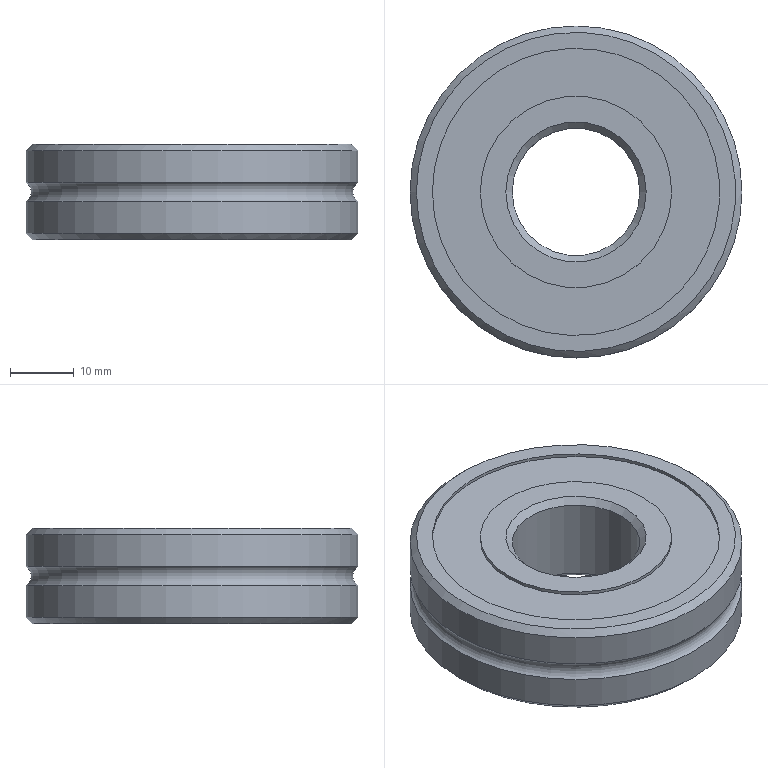Component | NX | BENT_SHAFT_2 | 1 solid | 18 faces | box 52 x 52 x 15 mm | volume 25760 mm3 | cylinder 7 | plane 6 | cone 4 | torus 1 | commonest cylinder face diameters 45 x2 30 x2 52 x2 20 x1
STEP:
#1=CARTESIAN_POINT('',(0.,0.,0.));
#2=DIRECTION('',(0.,0.,1.));
#3=DIRECTION('',(1.,0.,0.));
#4=AXIS2_PLACEMENT_3D('',#1,#2,#3);
#5=CARTESIAN_POINT('',(1437.632,1212.,804.574));
#6=VERTEX_POINT('',#5);
#7=CARTESIAN_POINT('',(1460.132,1212.,804.574));
#8=DIRECTION('',(0.,0.,-1.));
#9=DIRECTION('',(-1.,0.,0.));
#10=AXIS2_PLACEMENT_3D('',#7,#8,#9);
#11=CIRCLE('',#10,22.5);
#12=CARTESIAN_POINT('',(1435.132,1212.,804.574));
#13=DIRECTION('',(0.,0.,1.));
#14=DIRECTION('',(1.,0.,0.));
#15=AXIS2_PLACEMENT_3D('',#12,#13,#14);
#16=PLANE('',#15);
#17=CARTESIAN_POINT('',(2.5,0.));
#18=CARTESIAN_POINT('',(2.5,38.971));
#19=CARTESIAN_POINT('',(36.25,19.486));
#20=CARTESIAN_POINT('',(70.,0.));
#21=CARTESIAN_POINT('',(36.25,-19.486));
#22=CARTESIAN_POINT('',(2.5,-38.971));
#23=CARTESIAN_POINT('',(2.5,0.));
#24=(BOUNDED_CURVE()B_SPLINE_CURVE(2,(#17,#18,#19,#20,#21,#22,#23),.UNSPECIFIED.,.T.,.F.)B_SPLINE_CURVE_WITH_KNOTS((1,2,2,2,2,1),(-2.094,0.,2.094,4.189,6.283,8.378),.UNSPECIFIED.)CURVE()GEOMETRIC_REPRESENTATION_ITEM()RATIONAL_B_SPLINE_CURVE((1.,0.5,1.,0.5,1.,0.5,1.))REPRESENTATION_ITEM(''));
#25=(GEOMETRIC_REPRESENTATION_CONTEXT(2)PARAMETRIC_REPRESENTATION_CONTEXT()REPRESENTATION_CONTEXT('',''));
#26=DEFINITIONAL_REPRESENTATION('',(#24),#25);
#27=PCURVE('',#16,#26);
#28=CARTESIAN_POINT('',(1460.132,1212.,786.574));
#29=DIRECTION('',(0.,0.,-1.));
#30=DIRECTION('',(-1.,0.,0.));
#31=AXIS2_PLACEMENT_3D('',#28,#29,#30);
#32=CYLINDRICAL_SURFACE('',#31,22.5);
#33=CARTESIAN_POINT('',(0.,-18.));
#34=DIRECTION('',(1.,0.));
#35=VECTOR('',#34,1.);
#36=LINE('',#33,#35);
#37=(GEOMETRIC_REPRESENTATION_CONTEXT(2)PARAMETRIC_REPRESENTATION_CONTEXT()REPRESENTATION_CONTEXT('',''));
#38=DEFINITIONAL_REPRESENTATION('',(#36),#37);
#39=PCURVE('',#32,#38);
#40=SURFACE_CURVE('',#11,(#27,#39),.PCURVE_S1.);
#41=EDGE_CURVE('',#6,#6,#40,.T.);
#42=ORIENTED_EDGE('',*,*,#41,.F.);
#43=EDGE_LOOP('',(#42));
#44=FACE_BOUND('',#43,.T.);
#45=CARTESIAN_POINT('',(1435.132,1212.,804.574));
#46=VERTEX_POINT('',#45);
#47=CARTESIAN_POINT('',(1460.132,1212.,804.574));
#48=DIRECTION('',(0.,0.,-1.));
#49=DIRECTION('',(-1.,0.,0.));
#50=AXIS2_PLACEMENT_3D('',#47,#48,#49);
#51=CIRCLE('',#50,25.);
#52=CARTESIAN_POINT('',(0.,0.));
#53=CARTESIAN_POINT('',(0.,43.301));
#54=CARTESIAN_POINT('',(37.5,21.651));
#55=CARTESIAN_POINT('',(75.,0.));
#56=CARTESIAN_POINT('',(37.5,-21.651));
#57=CARTESIAN_POINT('',(0.,-43.301));
#58=CARTESIAN_POINT('',(0.,0.));
#59=(BOUNDED_CURVE()B_SPLINE_CURVE(2,(#52,#53,#54,#55,#56,#57,#58),.UNSPECIFIED.,.T.,.F.)B_SPLINE_CURVE_WITH_KNOTS((1,2,2,2,2,1),(-2.094,0.,2.094,4.189,6.283,8.378),.UNSPECIFIED.)CURVE()GEOMETRIC_REPRESENTATION_ITEM()RATIONAL_B_SPLINE_CURVE((1.,0.5,1.,0.5,1.,0.5,1.))REPRESENTATION_ITEM(''));
#60=(GEOMETRIC_REPRESENTATION_CONTEXT(2)PARAMETRIC_REPRESENTATION_CONTEXT()REPRESENTATION_CONTEXT('',''));
#61=DEFINITIONAL_REPRESENTATION('',(#59),#60);
#62=PCURVE('',#16,#61);
#63=CARTESIAN_POINT('',(1460.132,1212.,805.574));
#64=DIRECTION('',(0.,0.,1.));
#65=DIRECTION('',(1.,0.,0.));
#66=AXIS2_PLACEMENT_3D('',#63,#64,#65);
#67=CONICAL_SURFACE('',#66,26.,0.7854);
#68=CARTESIAN_POINT('',(9.425,-1.));
#69=DIRECTION('',(-1.,0.));
#70=VECTOR('',#69,1.);
#71=LINE('',#68,#70);
#72=(GEOMETRIC_REPRESENTATION_CONTEXT(2)PARAMETRIC_REPRESENTATION_CONTEXT()REPRESENTATION_CONTEXT('',''));
#73=DEFINITIONAL_REPRESENTATION('',(#71),#72);
#74=PCURVE('',#67,#73);
#75=SURFACE_CURVE('',#51,(#62,#74),.PCURVE_S1.);
#76=EDGE_CURVE('',#46,#46,#75,.T.);
#77=ORIENTED_EDGE('',*,*,#76,.T.);
#78=EDGE_LOOP('',(#77));
#79=FACE_BOUND('',#78,.T.);
#80=ADVANCED_FACE('',(#44,#79),#16,.F.);
#81=CARTESIAN_POINT('',(1437.632,1212.,805.074));
#82=VERTEX_POINT('',#81);
#83=CARTESIAN_POINT('',(1460.132,1212.,805.074));
#84=DIRECTION('',(0.,0.,-1.));
#85=DIRECTION('',(-1.,0.,0.));
#86=AXIS2_PLACEMENT_3D('',#83,#84,#85);
#87=CIRCLE('',#86,22.5);
#88=CARTESIAN_POINT('',(0.,-18.5));
#89=DIRECTION('',(1.,0.));
#90=VECTOR('',#89,1.);
#91=LINE('',#88,#90);
#92=(GEOMETRIC_REPRESENTATION_CONTEXT(2)PARAMETRIC_REPRESENTATION_CONTEXT()REPRESENTATION_CONTEXT('',''));
#93=DEFINITIONAL_REPRESENTATION('',(#91),#92);
#94=PCURVE('',#32,#93);
#95=CARTESIAN_POINT('',(1437.632,1212.,805.074));
#96=DIRECTION('',(0.,0.,1.));
#97=DIRECTION('',(1.,0.,0.));
#98=AXIS2_PLACEMENT_3D('',#95,#96,#97);
#99=PLANE('',#98);
#100=CARTESIAN_POINT('',(0.,0.));
#101=CARTESIAN_POINT('',(0.,38.971));
#102=CARTESIAN_POINT('',(33.75,19.486));
#103=CARTESIAN_POINT('',(67.5,0.));
#104=CARTESIAN_POINT('',(33.75,-19.486));
#105=CARTESIAN_POINT('',(0.,-38.971));
#106=CARTESIAN_POINT('',(0.,0.));
#107=(BOUNDED_CURVE()B_SPLINE_CURVE(2,(#100,#101,#102,#103,#104,#105,#106),.UNSPECIFIED.,.T.,.F.)B_SPLINE_CURVE_WITH_KNOTS((1,2,2,2,2,1),(-2.094,0.,2.094,4.189,6.283,8.378),.UNSPECIFIED.)CURVE()GEOMETRIC_REPRESENTATION_ITEM()RATIONAL_B_SPLINE_CURVE((1.,0.5,1.,0.5,1.,0.5,1.))REPRESENTATION_ITEM(''));
#108=(GEOMETRIC_REPRESENTATION_CONTEXT(2)PARAMETRIC_REPRESENTATION_CONTEXT()REPRESENTATION_CONTEXT('',''));
#109=DEFINITIONAL_REPRESENTATION('',(#107),#108);
#110=PCURVE('',#99,#109);
#111=SURFACE_CURVE('',#87,(#94,#110),.PCURVE_S1.);
#112=EDGE_CURVE('',#82,#82,#111,.T.);
#113=ORIENTED_EDGE('',*,*,#112,.T.);
#114=CARTESIAN_POINT('',(1437.632,1212.,805.074));
#115=CARTESIAN_POINT('',(1437.632,1212.,804.574));
#116=B_SPLINE_CURVE_WITH_KNOTS('',1,(#114,#115),.UNSPECIFIED.,.F.,.F.,(2,2),(-18.5,-18.),.PIECEWISE_BEZIER_KNOTS.);
#117=CARTESIAN_POINT('',(6.283,0.));
#118=DIRECTION('',(0.,1.));
#119=VECTOR('',#118,1.);
#120=LINE('',#117,#119);
#121=(GEOMETRIC_REPRESENTATION_CONTEXT(2)PARAMETRIC_REPRESENTATION_CONTEXT()REPRESENTATION_CONTEXT('',''));
#122=DEFINITIONAL_REPRESENTATION('',(#120),#121);
#123=PCURVE('',#32,#122);
#124=CARTESIAN_POINT('',(0.,0.));
#125=DIRECTION('',(0.,1.));
#126=VECTOR('',#125,1.);
#127=LINE('',#124,#126);
#128=(GEOMETRIC_REPRESENTATION_CONTEXT(2)PARAMETRIC_REPRESENTATION_CONTEXT()REPRESENTATION_CONTEXT('',''));
#129=DEFINITIONAL_REPRESENTATION('',(#127),#128);
#130=PCURVE('',#32,#129);
#131=SEAM_CURVE('',#116,(#123,#130),.PCURVE_S1.);
#132=EDGE_CURVE('',#82,#6,#131,.T.);
#133=ORIENTED_EDGE('',*,*,#132,.T.);
#134=ORIENTED_EDGE('',*,*,#41,.F.);
#135=ORIENTED_EDGE('',*,*,#132,.F.);
#136=EDGE_LOOP('',(#113,#133,#134,#135));
#137=FACE_BOUND('',#136,.F.);
#138=ADVANCED_FACE('',(#137),#32,.F.);
#139=CARTESIAN_POINT('',(1445.132,1212.,805.074));
#140=VERTEX_POINT('',#139);
#141=CARTESIAN_POINT('',(1460.132,1212.,805.074));
#142=DIRECTION('',(0.,0.,-1.));
#143=DIRECTION('',(-1.,0.,0.));
#144=AXIS2_PLACEMENT_3D('',#141,#142,#143);
#145=CIRCLE('',#144,15.);
#146=CARTESIAN_POINT('',(7.5,0.));
#147=CARTESIAN_POINT('',(7.5,25.981));
#148=CARTESIAN_POINT('',(30.,12.99));
#149=CARTESIAN_POINT('',(52.5,0.));
#150=CARTESIAN_POINT('',(30.,-12.99));
#151=CARTESIAN_POINT('',(7.5,-25.981));
#152=CARTESIAN_POINT('',(7.5,0.));
#153=(BOUNDED_CURVE()B_SPLINE_CURVE(2,(#146,#147,#148,#149,#150,#151,#152),.UNSPECIFIED.,.T.,.F.)B_SPLINE_CURVE_WITH_KNOTS((1,2,2,2,2,1),(-2.094,0.,2.094,4.189,6.283,8.378),.UNSPECIFIED.)CURVE()GEOMETRIC_REPRESENTATION_ITEM()RATIONAL_B_SPLINE_CURVE((1.,0.5,1.,0.5,1.,0.5,1.))REPRESENTATION_ITEM(''));
#154=(GEOMETRIC_REPRESENTATION_CONTEXT(2)PARAMETRIC_REPRESENTATION_CONTEXT()REPRESENTATION_CONTEXT('',''));
#155=DEFINITIONAL_REPRESENTATION('',(#153),#154);
#156=PCURVE('',#99,#155);
#157=CARTESIAN_POINT('',(1460.132,1212.,786.574));
#158=DIRECTION('',(0.,0.,-1.));
#159=DIRECTION('',(-1.,0.,0.));
#160=AXIS2_PLACEMENT_3D('',#157,#158,#159);
#161=CYLINDRICAL_SURFACE('',#160,15.);
#162=CARTESIAN_POINT('',(0.,-18.5));
#163=DIRECTION('',(1.,0.));
#164=VECTOR('',#163,1.);
#165=LINE('',#162,#164);
#166=(GEOMETRIC_REPRESENTATION_CONTEXT(2)PARAMETRIC_REPRESENTATION_CONTEXT()REPRESENTATION_CONTEXT('',''));
#167=DEFINITIONAL_REPRESENTATION('',(#165),#166);
#168=PCURVE('',#161,#167);
#169=SURFACE_CURVE('',#145,(#156,#168),.PCURVE_S1.);
#170=EDGE_CURVE('',#140,#140,#169,.T.);
#171=ORIENTED_EDGE('',*,*,#170,.F.);
#172=EDGE_LOOP('',(#171));
#173=FACE_BOUND('',#172,.T.);
#174=ORIENTED_EDGE('',*,*,#112,.T.);
#175=EDGE_LOOP('',(#174));
#176=FACE_BOUND('',#175,.T.);
#177=ADVANCED_FACE('',(#173,#176),#99,.F.);
#178=CARTESIAN_POINT('',(1445.132,1212.,804.574));
#179=VERTEX_POINT('',#178);
#180=CARTESIAN_POINT('',(1460.132,1212.,804.574));
#181=DIRECTION('',(0.,0.,-1.));
#182=DIRECTION('',(-1.,0.,0.));
#183=AXIS2_PLACEMENT_3D('',#180,#181,#182);
#184=CIRCLE('',#183,15.);
#185=CARTESIAN_POINT('',(0.,-18.));
#186=DIRECTION('',(1.,0.));
#187=VECTOR('',#186,1.);
#188=LINE('',#185,#187);
#189=(GEOMETRIC_REPRESENTATION_CONTEXT(2)PARAMETRIC_REPRESENTATION_CONTEXT()REPRESENTATION_CONTEXT('',''));
#190=DEFINITIONAL_REPRESENTATION('',(#188),#189);
#191=PCURVE('',#161,#190);
#192=CARTESIAN_POINT('',(1445.132,1212.,804.574));
#193=DIRECTION('',(0.,0.,1.));
#194=DIRECTION('',(1.,0.,0.));
#195=AXIS2_PLACEMENT_3D('',#192,#193,#194);
#196=PLANE('',#195);
#197=CARTESIAN_POINT('',(0.,0.));
#198=CARTESIAN_POINT('',(0.,25.981));
#199=CARTESIAN_POINT('',(22.5,12.99));
#200=CARTESIAN_POINT('',(45.,0.));
#201=CARTESIAN_POINT('',(22.5,-12.99));
#202=CARTESIAN_POINT('',(0.,-25.981));
#203=CARTESIAN_POINT('',(0.,0.));
#204=(BOUNDED_CURVE()B_SPLINE_CURVE(2,(#197,#198,#199,#200,#201,#202,#203),.UNSPECIFIED.,.T.,.F.)B_SPLINE_CURVE_WITH_KNOTS((1,2,2,2,2,1),(-2.094,0.,2.094,4.189,6.283,8.378),.UNSPECIFIED.)CURVE()GEOMETRIC_REPRESENTATION_ITEM()RATIONAL_B_SPLINE_CURVE((1.,0.5,1.,0.5,1.,0.5,1.))REPRESENTATION_ITEM(''));
#205=(GEOMETRIC_REPRESENTATION_CONTEXT(2)PARAMETRIC_REPRESENTATION_CONTEXT()REPRESENTATION_CONTEXT('',''));
#206=DEFINITIONAL_REPRESENTATION('',(#204),#205);
#207=PCURVE('',#196,#206);
#208=SURFACE_CURVE('',#184,(#191,#207),.PCURVE_S1.);
#209=EDGE_CURVE('',#179,#179,#208,.T.);
#210=ORIENTED_EDGE('',*,*,#209,.F.);
#211=CARTESIAN_POINT('',(1445.132,1212.,805.074));
#212=CARTESIAN_POINT('',(1445.132,1212.,804.574));
#213=B_SPLINE_CURVE_WITH_KNOTS('',1,(#211,#212),.UNSPECIFIED.,.F.,.F.,(2,2),(-18.5,-18.),.PIECEWISE_BEZIER_KNOTS.);
#214=CARTESIAN_POINT('',(0.,0.));
#215=DIRECTION('',(0.,1.));
#216=VECTOR('',#215,1.);
#217=LINE('',#214,#216);
#218=(GEOMETRIC_REPRESENTATION_CONTEXT(2)PARAMETRIC_REPRESENTATION_CONTEXT()REPRESENTATION_CONTEXT('',''));
#219=DEFINITIONAL_REPRESENTATION('',(#217),#218);
#220=PCURVE('',#161,#219);
#221=CARTESIAN_POINT('',(6.283,0.));
#222=DIRECTION('',(0.,1.));
#223=VECTOR('',#222,1.);
#224=LINE('',#221,#223);
#225=(GEOMETRIC_REPRESENTATION_CONTEXT(2)PARAMETRIC_REPRESENTATION_CONTEXT()REPRESENTATION_CONTEXT('',''));
#226=DEFINITIONAL_REPRESENTATION('',(#224),#225);
#227=PCURVE('',#161,#226);
#228=SEAM_CURVE('',#213,(#220,#227),.PCURVE_S1.);
#229=EDGE_CURVE('',#140,#179,#228,.T.);
#230=ORIENTED_EDGE('',*,*,#229,.F.);
#231=ORIENTED_EDGE('',*,*,#170,.T.);
#232=ORIENTED_EDGE('',*,*,#229,.T.);
#233=EDGE_LOOP('',(#210,#230,#231,#232));
#234=FACE_BOUND('',#233,.T.);
#235=ADVANCED_FACE('',(#234),#161,.T.);
#236=CARTESIAN_POINT('',(1471.132,1212.,804.574));
#237=VERTEX_POINT('',#236);
#238=CARTESIAN_POINT('',(1460.132,1212.,804.574));
#239=DIRECTION('',(0.,0.,1.));
#240=DIRECTION('',(1.,0.,0.));
#241=AXIS2_PLACEMENT_3D('',#238,#239,#240);
#242=CIRCLE('',#241,11.);
#243=CARTESIAN_POINT('',(15.,0.));
#244=DIRECTION('',(1.,0.));
#245=AXIS2_PLACEMENT_2D('',#243,#244);
#246=CIRCLE('',#245,11.);
#247=(GEOMETRIC_REPRESENTATION_CONTEXT(2)PARAMETRIC_REPRESENTATION_CONTEXT()REPRESENTATION_CONTEXT('',''));
#248=DEFINITIONAL_REPRESENTATION('',(#246),#247);
#249=PCURVE('',#196,#248);
#250=CARTESIAN_POINT('',(1460.132,1212.,805.574));
#251=DIRECTION('',(0.,0.,-1.));
#252=DIRECTION('',(-1.,0.,0.));
#253=AXIS2_PLACEMENT_3D('',#250,#251,#252);
#254=CONICAL_SURFACE('',#253,10.,0.7854);
#255=CARTESIAN_POINT('',(9.425,1.));
#256=DIRECTION('',(-1.,0.));
#257=VECTOR('',#256,1.);
#258=LINE('',#255,#257);
#259=(GEOMETRIC_REPRESENTATION_CONTEXT(2)PARAMETRIC_REPRESENTATION_CONTEXT()REPRESENTATION_CONTEXT('',''));
#260=DEFINITIONAL_REPRESENTATION('',(#258),#259);
#261=PCURVE('',#254,#260);
#262=SURFACE_CURVE('',#242,(#249,#261),.PCURVE_S1.);
#263=EDGE_CURVE('',#237,#237,#262,.T.);
#264=ORIENTED_EDGE('',*,*,#263,.T.);
#265=EDGE_LOOP('',(#264));
#266=FACE_BOUND('',#265,.T.);
#267=ORIENTED_EDGE('',*,*,#209,.T.);
#268=EDGE_LOOP('',(#267));
#269=FACE_BOUND('',#268,.T.);
#270=ADVANCED_FACE('',(#266,#269),#196,.F.);
#271=CARTESIAN_POINT('',(1450.132,1212.,818.574));
#272=VERTEX_POINT('',#271);
#273=CARTESIAN_POINT('',(1460.132,1212.,818.574));
#274=DIRECTION('',(0.,0.,1.));
#275=DIRECTION('',(-1.,0.,0.));
#276=AXIS2_PLACEMENT_3D('',#273,#274,#275);
#277=CIRCLE('',#276,10.);
#278=CARTESIAN_POINT('',(1460.132,1212.,786.574));
#279=DIRECTION('',(0.,0.,-1.));
#280=DIRECTION('',(-1.,0.,0.));
#281=AXIS2_PLACEMENT_3D('',#278,#279,#280);
#282=CYLINDRICAL_SURFACE('',#281,10.);
#283=CARTESIAN_POINT('',(6.283,-32.));
#284=DIRECTION('',(-1.,0.));
#285=VECTOR('',#284,1.);
#286=LINE('',#283,#285);
#287=(GEOMETRIC_REPRESENTATION_CONTEXT(2)PARAMETRIC_REPRESENTATION_CONTEXT()REPRESENTATION_CONTEXT('',''));
#288=DEFINITIONAL_REPRESENTATION('',(#286),#287);
#289=PCURVE('',#282,#288);
#290=CARTESIAN_POINT('',(1460.132,1212.,819.574));
#291=DIRECTION('',(0.,0.,1.));
#292=DIRECTION('',(1.,0.,0.));
#293=AXIS2_PLACEMENT_3D('',#290,#291,#292);
#294=CONICAL_SURFACE('',#293,11.,0.7854);
#295=CARTESIAN_POINT('',(3.142,-1.));
#296=DIRECTION('',(1.,0.));
#297=VECTOR('',#296,1.);
#298=LINE('',#295,#297);
#299=(GEOMETRIC_REPRESENTATION_CONTEXT(2)PARAMETRIC_REPRESENTATION_CONTEXT()REPRESENTATION_CONTEXT('',''));
#300=DEFINITIONAL_REPRESENTATION('',(#298),#299);
#301=PCURVE('',#294,#300);
#302=SURFACE_CURVE('',#277,(#289,#301),.PCURVE_S1.);
#303=EDGE_CURVE('',#272,#272,#302,.T.);
#304=ORIENTED_EDGE('',*,*,#303,.F.);
#305=CARTESIAN_POINT('',(1450.132,1212.,805.574));
#306=VERTEX_POINT('',#305);
#307=CARTESIAN_POINT('',(1450.132,1212.,818.574));
#308=CARTESIAN_POINT('',(1450.132,1212.,805.574));
#309=B_SPLINE_CURVE_WITH_KNOTS('',1,(#307,#308),.UNSPECIFIED.,.F.,.F.,(2,2),(-32.,-19.),.PIECEWISE_BEZIER_KNOTS.);
#310=CARTESIAN_POINT('',(6.283,0.));
#311=DIRECTION('',(0.,1.));
#312=VECTOR('',#311,1.);
#313=LINE('',#310,#312);
#314=(GEOMETRIC_REPRESENTATION_CONTEXT(2)PARAMETRIC_REPRESENTATION_CONTEXT()REPRESENTATION_CONTEXT('',''));
#315=DEFINITIONAL_REPRESENTATION('',(#313),#314);
#316=PCURVE('',#282,#315);
#317=CARTESIAN_POINT('',(0.,0.));
#318=DIRECTION('',(0.,1.));
#319=VECTOR('',#318,1.);
#320=LINE('',#317,#319);
#321=(GEOMETRIC_REPRESENTATION_CONTEXT(2)PARAMETRIC_REPRESENTATION_CONTEXT()REPRESENTATION_CONTEXT('',''));
#322=DEFINITIONAL_REPRESENTATION('',(#320),#321);
#323=PCURVE('',#282,#322);
#324=SEAM_CURVE('',#309,(#316,#323),.PCURVE_S1.);
#325=EDGE_CURVE('',#272,#306,#324,.T.);
#326=ORIENTED_EDGE('',*,*,#325,.T.);
#327=CARTESIAN_POINT('',(1470.132,1212.,805.574));
#328=VERTEX_POINT('',#327);
#329=CARTESIAN_POINT('',(1460.132,1212.,805.574));
#330=DIRECTION('',(0.,0.,-1.));
#331=DIRECTION('',(1.,0.,0.));
#332=AXIS2_PLACEMENT_3D('',#329,#330,#331);
#333=CIRCLE('',#332,10.);
#334=CARTESIAN_POINT('',(3.142,-19.));
#335=DIRECTION('',(1.,0.));
#336=VECTOR('',#335,1.);
#337=LINE('',#334,#336);
#338=(GEOMETRIC_REPRESENTATION_CONTEXT(2)PARAMETRIC_REPRESENTATION_CONTEXT()REPRESENTATION_CONTEXT('',''));
#339=DEFINITIONAL_REPRESENTATION('',(#337),#338);
#340=PCURVE('',#282,#339);
#341=CARTESIAN_POINT('',(3.142,-0.));
#342=DIRECTION('',(1.,0.));
#343=VECTOR('',#342,1.);
#344=LINE('',#341,#343);
#345=(GEOMETRIC_REPRESENTATION_CONTEXT(2)PARAMETRIC_REPRESENTATION_CONTEXT()REPRESENTATION_CONTEXT('',''));
#346=DEFINITIONAL_REPRESENTATION('',(#344),#345);
#347=PCURVE('',#254,#346);
#348=SURFACE_CURVE('',#333,(#340,#347),.PCURVE_S1.);
#349=EDGE_CURVE('',#328,#306,#348,.T.);
#350=ORIENTED_EDGE('',*,*,#349,.F.);
#351=CARTESIAN_POINT('',(1460.132,1212.,805.574));
#352=DIRECTION('',(0.,0.,-1.));
#353=DIRECTION('',(1.,0.,0.));
#354=AXIS2_PLACEMENT_3D('',#351,#352,#353);
#355=CIRCLE('',#354,10.);
#356=CARTESIAN_POINT('',(-3.142,-19.));
#357=DIRECTION('',(1.,0.));
#358=VECTOR('',#357,1.);
#359=LINE('',#356,#358);
#360=(GEOMETRIC_REPRESENTATION_CONTEXT(2)PARAMETRIC_REPRESENTATION_CONTEXT()REPRESENTATION_CONTEXT('',''));
#361=DEFINITIONAL_REPRESENTATION('',(#359),#360);
#362=PCURVE('',#282,#361);
#363=CARTESIAN_POINT('',(3.142,-0.));
#364=DIRECTION('',(1.,0.));
#365=VECTOR('',#364,1.);
#366=LINE('',#363,#365);
#367=(GEOMETRIC_REPRESENTATION_CONTEXT(2)PARAMETRIC_REPRESENTATION_CONTEXT()REPRESENTATION_CONTEXT('',''));
#368=DEFINITIONAL_REPRESENTATION('',(#366),#367);
#369=PCURVE('',#254,#368);
#370=SURFACE_CURVE('',#355,(#362,#369),.PCURVE_S1.);
#371=EDGE_CURVE('',#306,#328,#370,.T.);
#372=ORIENTED_EDGE('',*,*,#371,.F.);
#373=ORIENTED_EDGE('',*,*,#325,.F.);
#374=EDGE_LOOP('',(#304,#326,#350,#372,#373));
#375=FACE_BOUND('',#374,.F.);
#376=ADVANCED_FACE('',(#375),#282,.F.);
#377=CARTESIAN_POINT('',(1449.132,1212.,819.574));
#378=VERTEX_POINT('',#377);
#379=CARTESIAN_POINT('',(1460.132,1212.,819.574));
#380=DIRECTION('',(0.,0.,-1.));
#381=DIRECTION('',(-1.,0.,0.));
#382=AXIS2_PLACEMENT_3D('',#379,#380,#381);
#383=CIRCLE('',#382,11.);
#384=CARTESIAN_POINT('',(1450.132,1212.,819.574));
#385=DIRECTION('',(0.,0.,-1.));
#386=DIRECTION('',(-1.,0.,0.));
#387=AXIS2_PLACEMENT_3D('',#384,#385,#386);
#388=PLANE('',#387);
#389=CARTESIAN_POINT('',(-10.,0.));
#390=DIRECTION('',(1.,0.));
#391=AXIS2_PLACEMENT_2D('',#389,#390);
#392=CIRCLE('',#391,11.);
#393=(GEOMETRIC_REPRESENTATION_CONTEXT(2)PARAMETRIC_REPRESENTATION_CONTEXT()REPRESENTATION_CONTEXT('',''));
#394=DEFINITIONAL_REPRESENTATION('',(#392),#393);
#395=PCURVE('',#388,#394);
#396=CARTESIAN_POINT('',(9.425,0.));
#397=DIRECTION('',(-1.,0.));
#398=VECTOR('',#397,1.);
#399=LINE('',#396,#398);
#400=(GEOMETRIC_REPRESENTATION_CONTEXT(2)PARAMETRIC_REPRESENTATION_CONTEXT()REPRESENTATION_CONTEXT('',''));
#401=DEFINITIONAL_REPRESENTATION('',(#399),#400);
#402=PCURVE('',#294,#401);
#403=SURFACE_CURVE('',#383,(#395,#402),.PCURVE_S1.);
#404=EDGE_CURVE('',#378,#378,#403,.T.);
#405=ORIENTED_EDGE('',*,*,#404,.T.);
#406=EDGE_LOOP('',(#405));
#407=FACE_BOUND('',#406,.T.);
#408=CARTESIAN_POINT('',(1445.132,1212.,819.574));
#409=VERTEX_POINT('',#408);
#410=CARTESIAN_POINT('',(1460.132,1212.,819.574));
#411=DIRECTION('',(0.,0.,-1.));
#412=DIRECTION('',(-1.,0.,0.));
#413=AXIS2_PLACEMENT_3D('',#410,#411,#412);
#414=CIRCLE('',#413,15.);
#415=CARTESIAN_POINT('',(-10.,0.));
#416=DIRECTION('',(1.,0.));
#417=AXIS2_PLACEMENT_2D('',#415,#416);
#418=CIRCLE('',#417,15.);
#419=(GEOMETRIC_REPRESENTATION_CONTEXT(2)PARAMETRIC_REPRESENTATION_CONTEXT()REPRESENTATION_CONTEXT('',''));
#420=DEFINITIONAL_REPRESENTATION('',(#418),#419);
#421=PCURVE('',#388,#420);
#422=CARTESIAN_POINT('',(1460.132,1212.,786.574));
#423=DIRECTION('',(0.,0.,-1.));
#424=DIRECTION('',(-1.,0.,0.));
#425=AXIS2_PLACEMENT_3D('',#422,#423,#424);
#426=CYLINDRICAL_SURFACE('',#425,15.);
#427=CARTESIAN_POINT('',(0.,-33.));
#428=DIRECTION('',(1.,0.));
#429=VECTOR('',#428,1.);
#430=LINE('',#427,#429);
#431=(GEOMETRIC_REPRESENTATION_CONTEXT(2)PARAMETRIC_REPRESENTATION_CONTEXT()REPRESENTATION_CONTEXT('',''));
#432=DEFINITIONAL_REPRESENTATION('',(#430),#431);
#433=PCURVE('',#426,#432);
#434=SURFACE_CURVE('',#414,(#421,#433),.PCURVE_S1.);
#435=EDGE_CURVE('',#409,#409,#434,.T.);
#436=ORIENTED_EDGE('',*,*,#435,.F.);
#437=EDGE_LOOP('',(#436));
#438=FACE_BOUND('',#437,.T.);
#439=ADVANCED_FACE('',(#407,#438),#388,.F.);
#440=CARTESIAN_POINT('',(1445.132,1212.,819.074));
#441=VERTEX_POINT('',#440);
#442=CARTESIAN_POINT('',(1460.132,1212.,819.074));
#443=DIRECTION('',(0.,0.,-1.));
#444=DIRECTION('',(-1.,0.,0.));
#445=AXIS2_PLACEMENT_3D('',#442,#443,#444);
#446=CIRCLE('',#445,15.);
#447=CARTESIAN_POINT('',(0.,-32.5));
#448=DIRECTION('',(1.,0.));
#449=VECTOR('',#448,1.);
#450=LINE('',#447,#449);
#451=(GEOMETRIC_REPRESENTATION_CONTEXT(2)PARAMETRIC_REPRESENTATION_CONTEXT()REPRESENTATION_CONTEXT('',''));
#452=DEFINITIONAL_REPRESENTATION('',(#450),#451);
#453=PCURVE('',#426,#452);
#454=CARTESIAN_POINT('',(1445.132,1212.,819.074));
#455=DIRECTION('',(0.,0.,-1.));
#456=DIRECTION('',(-1.,0.,0.));
#457=AXIS2_PLACEMENT_3D('',#454,#455,#456);
#458=PLANE('',#457);
#459=CARTESIAN_POINT('',(-15.,0.));
#460=DIRECTION('',(1.,0.));
#461=AXIS2_PLACEMENT_2D('',#459,#460);
#462=CIRCLE('',#461,15.);
#463=(GEOMETRIC_REPRESENTATION_CONTEXT(2)PARAMETRIC_REPRESENTATION_CONTEXT()REPRESENTATION_CONTEXT('',''));
#464=DEFINITIONAL_REPRESENTATION('',(#462),#463);
#465=PCURVE('',#458,#464);
#466=SURFACE_CURVE('',#446,(#453,#465),.PCURVE_S1.);
#467=EDGE_CURVE('',#441,#441,#466,.T.);
#468=ORIENTED_EDGE('',*,*,#467,.F.);
#469=CARTESIAN_POINT('',(1445.132,1212.,819.574));
#470=CARTESIAN_POINT('',(1445.132,1212.,819.074));
#471=B_SPLINE_CURVE_WITH_KNOTS('',1,(#469,#470),.UNSPECIFIED.,.F.,.F.,(2,2),(-33.,-32.5),.PIECEWISE_BEZIER_KNOTS.);
#472=CARTESIAN_POINT('',(0.,0.));
#473=DIRECTION('',(0.,1.));
#474=VECTOR('',#473,1.);
#475=LINE('',#472,#474);
#476=(GEOMETRIC_REPRESENTATION_CONTEXT(2)PARAMETRIC_REPRESENTATION_CONTEXT()REPRESENTATION_CONTEXT('',''));
#477=DEFINITIONAL_REPRESENTATION('',(#475),#476);
#478=PCURVE('',#426,#477);
#479=CARTESIAN_POINT('',(6.283,0.));
#480=DIRECTION('',(0.,1.));
#481=VECTOR('',#480,1.);
#482=LINE('',#479,#481);
#483=(GEOMETRIC_REPRESENTATION_CONTEXT(2)PARAMETRIC_REPRESENTATION_CONTEXT()REPRESENTATION_CONTEXT('',''));
#484=DEFINITIONAL_REPRESENTATION('',(#482),#483);
#485=PCURVE('',#426,#484);
#486=SEAM_CURVE('',#471,(#478,#485),.PCURVE_S1.);
#487=EDGE_CURVE('',#409,#441,#486,.T.);
#488=ORIENTED_EDGE('',*,*,#487,.F.);
#489=ORIENTED_EDGE('',*,*,#435,.T.);
#490=ORIENTED_EDGE('',*,*,#487,.T.);
#491=EDGE_LOOP('',(#468,#488,#489,#490));
#492=FACE_BOUND('',#491,.T.);
#493=ADVANCED_FACE('',(#492),#426,.T.);
#494=CARTESIAN_POINT('',(1437.632,1212.,819.074));
#495=VERTEX_POINT('',#494);
#496=CARTESIAN_POINT('',(1460.132,1212.,819.074));
#497=DIRECTION('',(0.,0.,-1.));
#498=DIRECTION('',(-1.,0.,0.));
#499=AXIS2_PLACEMENT_3D('',#496,#497,#498);
#500=CIRCLE('',#499,22.5);
#501=CARTESIAN_POINT('',(-15.,0.));
#502=DIRECTION('',(1.,0.));
#503=AXIS2_PLACEMENT_2D('',#501,#502);
#504=CIRCLE('',#503,22.5);
#505=(GEOMETRIC_REPRESENTATION_CONTEXT(2)PARAMETRIC_REPRESENTATION_CONTEXT()REPRESENTATION_CONTEXT('',''));
#506=DEFINITIONAL_REPRESENTATION('',(#504),#505);
#507=PCURVE('',#458,#506);
#508=CARTESIAN_POINT('',(1460.132,1212.,786.574));
#509=DIRECTION('',(0.,0.,-1.));
#510=DIRECTION('',(-1.,0.,0.));
#511=AXIS2_PLACEMENT_3D('',#508,#509,#510);
#512=CYLINDRICAL_SURFACE('',#511,22.5);
#513=CARTESIAN_POINT('',(0.,-32.5));
#514=DIRECTION('',(1.,0.));
#515=VECTOR('',#514,1.);
#516=LINE('',#513,#515);
#517=(GEOMETRIC_REPRESENTATION_CONTEXT(2)PARAMETRIC_REPRESENTATION_CONTEXT()REPRESENTATION_CONTEXT('',''));
#518=DEFINITIONAL_REPRESENTATION('',(#516),#517);
#519=PCURVE('',#512,#518);
#520=SURFACE_CURVE('',#500,(#507,#519),.PCURVE_S1.);
#521=EDGE_CURVE('',#495,#495,#520,.T.);
#522=ORIENTED_EDGE('',*,*,#521,.F.);
#523=EDGE_LOOP('',(#522));
#524=FACE_BOUND('',#523,.T.);
#525=ORIENTED_EDGE('',*,*,#467,.T.);
#526=EDGE_LOOP('',(#525));
#527=FACE_BOUND('',#526,.T.);
#528=ADVANCED_FACE('',(#524,#527),#458,.F.);
#529=CARTESIAN_POINT('',(1437.632,1212.,819.574));
#530=VERTEX_POINT('',#529);
#531=CARTESIAN_POINT('',(1460.132,1212.,819.574));
#532=DIRECTION('',(0.,0.,-1.));
#533=DIRECTION('',(-1.,0.,0.));
#534=AXIS2_PLACEMENT_3D('',#531,#532,#533);
#535=CIRCLE('',#534,22.5);
#536=CARTESIAN_POINT('',(0.,-33.));
#537=DIRECTION('',(1.,0.));
#538=VECTOR('',#537,1.);
#539=LINE('',#536,#538);
#540=(GEOMETRIC_REPRESENTATION_CONTEXT(2)PARAMETRIC_REPRESENTATION_CONTEXT()REPRESENTATION_CONTEXT('',''));
#541=DEFINITIONAL_REPRESENTATION('',(#539),#540);
#542=PCURVE('',#512,#541);
#543=CARTESIAN_POINT('',(1437.632,1212.,819.574));
#544=DIRECTION('',(0.,0.,-1.));
#545=DIRECTION('',(-1.,0.,0.));
#546=AXIS2_PLACEMENT_3D('',#543,#544,#545);
#547=PLANE('',#546);
#548=CARTESIAN_POINT('',(-22.5,0.));
#549=DIRECTION('',(1.,0.));
#550=AXIS2_PLACEMENT_2D('',#548,#549);
#551=CIRCLE('',#550,22.5);
#552=(GEOMETRIC_REPRESENTATION_CONTEXT(2)PARAMETRIC_REPRESENTATION_CONTEXT()REPRESENTATION_CONTEXT('',''));
#553=DEFINITIONAL_REPRESENTATION('',(#551),#552);
#554=PCURVE('',#547,#553);
#555=SURFACE_CURVE('',#535,(#542,#554),.PCURVE_S1.);
#556=EDGE_CURVE('',#530,#530,#555,.T.);
#557=ORIENTED_EDGE('',*,*,#556,.T.);
#558=CARTESIAN_POINT('',(1437.632,1212.,819.574));
#559=CARTESIAN_POINT('',(1437.632,1212.,819.074));
#560=B_SPLINE_CURVE_WITH_KNOTS('',1,(#558,#559),.UNSPECIFIED.,.F.,.F.,(2,2),(-33.,-32.5),.PIECEWISE_BEZIER_KNOTS.);
#561=CARTESIAN_POINT('',(6.283,0.));
#562=DIRECTION('',(0.,1.));
#563=VECTOR('',#562,1.);
#564=LINE('',#561,#563);
#565=(GEOMETRIC_REPRESENTATION_CONTEXT(2)PARAMETRIC_REPRESENTATION_CONTEXT()REPRESENTATION_CONTEXT('',''));
#566=DEFINITIONAL_REPRESENTATION('',(#564),#565);
#567=PCURVE('',#512,#566);
#568=CARTESIAN_POINT('',(0.,0.));
#569=DIRECTION('',(0.,1.));
#570=VECTOR('',#569,1.);
#571=LINE('',#568,#570);
#572=(GEOMETRIC_REPRESENTATION_CONTEXT(2)PARAMETRIC_REPRESENTATION_CONTEXT()REPRESENTATION_CONTEXT('',''));
#573=DEFINITIONAL_REPRESENTATION('',(#571),#572);
#574=PCURVE('',#512,#573);
#575=SEAM_CURVE('',#560,(#567,#574),.PCURVE_S1.);
#576=EDGE_CURVE('',#530,#495,#575,.T.);
#577=ORIENTED_EDGE('',*,*,#576,.T.);
#578=ORIENTED_EDGE('',*,*,#521,.F.);
#579=ORIENTED_EDGE('',*,*,#576,.F.);
#580=EDGE_LOOP('',(#557,#577,#578,#579));
#581=FACE_BOUND('',#580,.F.);
#582=ADVANCED_FACE('',(#581),#512,.F.);
#583=CARTESIAN_POINT('',(1435.132,1212.,819.574));
#584=VERTEX_POINT('',#583);
#585=CARTESIAN_POINT('',(1460.132,1212.,819.574));
#586=DIRECTION('',(0.,0.,-1.));
#587=DIRECTION('',(-1.,0.,0.));
#588=AXIS2_PLACEMENT_3D('',#585,#586,#587);
#589=CIRCLE('',#588,25.);
#590=CARTESIAN_POINT('',(-22.5,0.));
#591=DIRECTION('',(1.,0.));
#592=AXIS2_PLACEMENT_2D('',#590,#591);
#593=CIRCLE('',#592,25.);
#594=(GEOMETRIC_REPRESENTATION_CONTEXT(2)PARAMETRIC_REPRESENTATION_CONTEXT()REPRESENTATION_CONTEXT('',''));
#595=DEFINITIONAL_REPRESENTATION('',(#593),#594);
#596=PCURVE('',#547,#595);
#597=CARTESIAN_POINT('',(1460.132,1212.,819.574));
#598=DIRECTION('',(0.,0.,-1.));
#599=DIRECTION('',(-1.,0.,0.));
#600=AXIS2_PLACEMENT_3D('',#597,#598,#599);
#601=CONICAL_SURFACE('',#600,25.,0.7854);
#602=CARTESIAN_POINT('',(0.,0.));
#603=DIRECTION('',(1.,0.));
#604=VECTOR('',#603,1.);
#605=LINE('',#602,#604);
#606=(GEOMETRIC_REPRESENTATION_CONTEXT(2)PARAMETRIC_REPRESENTATION_CONTEXT()REPRESENTATION_CONTEXT('',''));
#607=DEFINITIONAL_REPRESENTATION('',(#605),#606);
#608=PCURVE('',#601,#607);
#609=SURFACE_CURVE('',#589,(#596,#608),.PCURVE_S1.);
#610=EDGE_CURVE('',#584,#584,#609,.T.);
#611=ORIENTED_EDGE('',*,*,#610,.F.);
#612=EDGE_LOOP('',(#611));
#613=FACE_BOUND('',#612,.T.);
#614=ORIENTED_EDGE('',*,*,#556,.T.);
#615=EDGE_LOOP('',(#614));
#616=FACE_BOUND('',#615,.T.);
#617=ADVANCED_FACE('',(#613,#616),#547,.F.);
#618=CARTESIAN_POINT('',(1434.132,1212.,818.574));
#619=VERTEX_POINT('',#618);
#620=CARTESIAN_POINT('',(1460.132,1212.,818.574));
#621=DIRECTION('',(0.,0.,-1.));
#622=DIRECTION('',(-1.,0.,0.));
#623=AXIS2_PLACEMENT_3D('',#620,#621,#622);
#624=CIRCLE('',#623,26.);
#625=CARTESIAN_POINT('',(0.,1.));
#626=DIRECTION('',(1.,0.));
#627=VECTOR('',#626,1.);
#628=LINE('',#625,#627);
#629=(GEOMETRIC_REPRESENTATION_CONTEXT(2)PARAMETRIC_REPRESENTATION_CONTEXT()REPRESENTATION_CONTEXT('',''));
#630=DEFINITIONAL_REPRESENTATION('',(#628),#629);
#631=PCURVE('',#601,#630);
#632=CARTESIAN_POINT('',(1460.132,1212.,786.574));
#633=DIRECTION('',(0.,0.,-1.));
#634=DIRECTION('',(-1.,0.,0.));
#635=AXIS2_PLACEMENT_3D('',#632,#633,#634);
#636=CYLINDRICAL_SURFACE('',#635,26.);
#637=CARTESIAN_POINT('',(0.,-32.));
#638=DIRECTION('',(1.,0.));
#639=VECTOR('',#638,1.);
#640=LINE('',#637,#639);
#641=(GEOMETRIC_REPRESENTATION_CONTEXT(2)PARAMETRIC_REPRESENTATION_CONTEXT()REPRESENTATION_CONTEXT('',''));
#642=DEFINITIONAL_REPRESENTATION('',(#640),#641);
#643=PCURVE('',#636,#642);
#644=SURFACE_CURVE('',#624,(#631,#643),.PCURVE_S1.);
#645=EDGE_CURVE('',#619,#619,#644,.T.);
#646=ORIENTED_EDGE('',*,*,#645,.F.);
#647=CARTESIAN_POINT('',(1435.132,1212.,819.574));
#648=CARTESIAN_POINT('',(1434.132,1212.,818.574));
#649=B_SPLINE_CURVE_WITH_KNOTS('',1,(#647,#648),.UNSPECIFIED.,.F.,.F.,(2,2),(0.,1.414),.PIECEWISE_BEZIER_KNOTS.);
#650=CARTESIAN_POINT('',(0.,0.));
#651=DIRECTION('',(0.,1.));
#652=VECTOR('',#651,1.);
#653=LINE('',#650,#652);
#654=(GEOMETRIC_REPRESENTATION_CONTEXT(2)PARAMETRIC_REPRESENTATION_CONTEXT()REPRESENTATION_CONTEXT('',''));
#655=DEFINITIONAL_REPRESENTATION('',(#653),#654);
#656=PCURVE('',#601,#655);
#657=CARTESIAN_POINT('',(6.283,0.));
#658=DIRECTION('',(0.,1.));
#659=VECTOR('',#658,1.);
#660=LINE('',#657,#659);
#661=(GEOMETRIC_REPRESENTATION_CONTEXT(2)PARAMETRIC_REPRESENTATION_CONTEXT()REPRESENTATION_CONTEXT('',''));
#662=DEFINITIONAL_REPRESENTATION('',(#660),#661);
#663=PCURVE('',#601,#662);
#664=SEAM_CURVE('',#649,(#656,#663),.PCURVE_S1.);
#665=EDGE_CURVE('',#584,#619,#664,.T.);
#666=ORIENTED_EDGE('',*,*,#665,.F.);
#667=ORIENTED_EDGE('',*,*,#610,.T.);
#668=ORIENTED_EDGE('',*,*,#665,.T.);
#669=EDGE_LOOP('',(#646,#666,#667,#668));
#670=FACE_BOUND('',#669,.T.);
#671=ADVANCED_FACE('',(#670),#601,.T.);
#672=CARTESIAN_POINT('',(1434.132,1212.,813.574));
#673=VERTEX_POINT('',#672);
#674=CARTESIAN_POINT('',(1460.132,1212.,813.574));
#675=DIRECTION('',(0.,0.,-1.));
#676=DIRECTION('',(-1.,0.,0.));
#677=AXIS2_PLACEMENT_3D('',#674,#675,#676);
#678=CIRCLE('',#677,26.);
#679=CARTESIAN_POINT('',(0.,-27.));
#680=DIRECTION('',(1.,0.));
#681=VECTOR('',#680,1.);
#682=LINE('',#679,#681);
#683=(GEOMETRIC_REPRESENTATION_CONTEXT(2)PARAMETRIC_REPRESENTATION_CONTEXT()REPRESENTATION_CONTEXT('',''));
#684=DEFINITIONAL_REPRESENTATION('',(#682),#683);
#685=PCURVE('',#636,#684);
#686=CARTESIAN_POINT('',(1460.132,1212.,812.074));
#687=DIRECTION('',(0.,0.,-1.));
#688=DIRECTION('',(-1.,0.,0.));
#689=AXIS2_PLACEMENT_3D('',#686,#687,#688);
#690=TOROIDAL_SURFACE('',#689,26.995,1.8);
#691=CARTESIAN_POINT('',(0.,4.127));
#692=DIRECTION('',(1.,0.));
#693=VECTOR('',#692,1.);
#694=LINE('',#691,#693);
#695=(GEOMETRIC_REPRESENTATION_CONTEXT(2)PARAMETRIC_REPRESENTATION_CONTEXT()REPRESENTATION_CONTEXT('',''));
#696=DEFINITIONAL_REPRESENTATION('',(#694),#695);
#697=PCURVE('',#690,#696);
#698=SURFACE_CURVE('',#678,(#685,#697),.PCURVE_S1.);
#699=EDGE_CURVE('',#673,#673,#698,.T.);
#700=ORIENTED_EDGE('',*,*,#699,.F.);
#701=CARTESIAN_POINT('',(1434.132,1212.,818.574));
#702=CARTESIAN_POINT('',(1434.132,1212.,813.574));
#703=B_SPLINE_CURVE_WITH_KNOTS('',1,(#701,#702),.UNSPECIFIED.,.F.,.F.,(2,2),(-32.,-27.),.PIECEWISE_BEZIER_KNOTS.);
#704=CARTESIAN_POINT('',(0.,0.));
#705=DIRECTION('',(0.,1.));
#706=VECTOR('',#705,1.);
#707=LINE('',#704,#706);
#708=(GEOMETRIC_REPRESENTATION_CONTEXT(2)PARAMETRIC_REPRESENTATION_CONTEXT()REPRESENTATION_CONTEXT('',''));
#709=DEFINITIONAL_REPRESENTATION('',(#707),#708);
#710=PCURVE('',#636,#709);
#711=CARTESIAN_POINT('',(6.283,0.));
#712=DIRECTION('',(0.,1.));
#713=VECTOR('',#712,1.);
#714=LINE('',#711,#713);
#715=(GEOMETRIC_REPRESENTATION_CONTEXT(2)PARAMETRIC_REPRESENTATION_CONTEXT()REPRESENTATION_CONTEXT('',''));
#716=DEFINITIONAL_REPRESENTATION('',(#714),#715);
#717=PCURVE('',#636,#716);
#718=SEAM_CURVE('',#703,(#710,#717),.PCURVE_S1.);
#719=EDGE_CURVE('',#619,#673,#718,.T.);
#720=ORIENTED_EDGE('',*,*,#719,.F.);
#721=ORIENTED_EDGE('',*,*,#645,.T.);
#722=ORIENTED_EDGE('',*,*,#719,.T.);
#723=EDGE_LOOP('',(#700,#720,#721,#722));
#724=FACE_BOUND('',#723,.T.);
#725=ADVANCED_FACE('',(#724),#636,.T.);
#726=CARTESIAN_POINT('',(1434.132,1212.,810.574));
#727=VERTEX_POINT('',#726);
#728=CARTESIAN_POINT('',(1460.132,1212.,810.574));
#729=DIRECTION('',(0.,0.,-1.));
#730=DIRECTION('',(-1.,0.,0.));
#731=AXIS2_PLACEMENT_3D('',#728,#729,#730);
#732=CIRCLE('',#731,26.);
#733=CARTESIAN_POINT('',(0.,2.156));
#734=DIRECTION('',(1.,0.));
#735=VECTOR('',#734,1.);
#736=LINE('',#733,#735);
#737=(GEOMETRIC_REPRESENTATION_CONTEXT(2)PARAMETRIC_REPRESENTATION_CONTEXT()REPRESENTATION_CONTEXT('',''));
#738=DEFINITIONAL_REPRESENTATION('',(#736),#737);
#739=PCURVE('',#690,#738);
#740=CARTESIAN_POINT('',(1460.132,1212.,786.574));
#741=DIRECTION('',(0.,0.,-1.));
#742=DIRECTION('',(-1.,0.,0.));
#743=AXIS2_PLACEMENT_3D('',#740,#741,#742);
#744=CYLINDRICAL_SURFACE('',#743,26.);
#745=CARTESIAN_POINT('',(0.,-24.));
#746=DIRECTION('',(1.,0.));
#747=VECTOR('',#746,1.);
#748=LINE('',#745,#747);
#749=(GEOMETRIC_REPRESENTATION_CONTEXT(2)PARAMETRIC_REPRESENTATION_CONTEXT()REPRESENTATION_CONTEXT('',''));
#750=DEFINITIONAL_REPRESENTATION('',(#748),#749);
#751=PCURVE('',#744,#750);
#752=SURFACE_CURVE('',#732,(#739,#751),.PCURVE_S1.);
#753=EDGE_CURVE('',#727,#727,#752,.T.);
#754=ORIENTED_EDGE('',*,*,#753,.T.);
#755=CARTESIAN_POINT('',(1434.132,1212.,810.574));
#756=CARTESIAN_POINT('',(1434.641,1212.,810.911));
#757=CARTESIAN_POINT('',(1434.994,1212.,811.439));
#758=CARTESIAN_POINT('',(1435.12,1212.,812.074));
#759=CARTESIAN_POINT('',(1434.994,1212.,812.708));
#760=CARTESIAN_POINT('',(1434.641,1212.,813.236));
#761=CARTESIAN_POINT('',(1434.132,1212.,813.574));
#762=(BOUNDED_CURVE()B_SPLINE_CURVE(6,(#755,#756,#757,#758,#759,#760,#761),.UNSPECIFIED.,.F.,.F.)B_SPLINE_CURVE_WITH_KNOTS((7,7),(2.156,4.127),.PIECEWISE_BEZIER_KNOTS.)CURVE()GEOMETRIC_REPRESENTATION_ITEM()RATIONAL_B_SPLINE_CURVE((1.05,1.016,0.9967,0.9906,0.9967,1.016,1.05))REPRESENTATION_ITEM(''));
#763=CARTESIAN_POINT('',(6.283,0.));
#764=DIRECTION('',(0.,1.));
#765=VECTOR('',#764,1.);
#766=LINE('',#763,#765);
#767=(GEOMETRIC_REPRESENTATION_CONTEXT(2)PARAMETRIC_REPRESENTATION_CONTEXT()REPRESENTATION_CONTEXT('',''));
#768=DEFINITIONAL_REPRESENTATION('',(#766),#767);
#769=PCURVE('',#690,#768);
#770=CARTESIAN_POINT('',(0.,0.));
#771=DIRECTION('',(0.,1.));
#772=VECTOR('',#771,1.);
#773=LINE('',#770,#772);
#774=(GEOMETRIC_REPRESENTATION_CONTEXT(2)PARAMETRIC_REPRESENTATION_CONTEXT()REPRESENTATION_CONTEXT('',''));
#775=DEFINITIONAL_REPRESENTATION('',(#773),#774);
#776=PCURVE('',#690,#775);
#777=SEAM_CURVE('',#762,(#769,#776),.PCURVE_S1.);
#778=EDGE_CURVE('',#727,#673,#777,.T.);
#779=ORIENTED_EDGE('',*,*,#778,.T.);
#780=ORIENTED_EDGE('',*,*,#699,.F.);
#781=ORIENTED_EDGE('',*,*,#778,.F.);
#782=EDGE_LOOP('',(#754,#779,#780,#781));
#783=FACE_BOUND('',#782,.F.);
#784=ADVANCED_FACE('',(#783),#690,.F.);
#785=CARTESIAN_POINT('',(1434.132,1212.,805.574));
#786=VERTEX_POINT('',#785);
#787=CARTESIAN_POINT('',(1460.132,1212.,805.574));
#788=DIRECTION('',(0.,0.,-1.));
#789=DIRECTION('',(-1.,0.,0.));
#790=AXIS2_PLACEMENT_3D('',#787,#788,#789);
#791=CIRCLE('',#790,26.);
#792=CARTESIAN_POINT('',(0.,-19.));
#793=DIRECTION('',(1.,0.));
#794=VECTOR('',#793,1.);
#795=LINE('',#792,#794);
#796=(GEOMETRIC_REPRESENTATION_CONTEXT(2)PARAMETRIC_REPRESENTATION_CONTEXT()REPRESENTATION_CONTEXT('',''));
#797=DEFINITIONAL_REPRESENTATION('',(#795),#796);
#798=PCURVE('',#744,#797);
#799=CARTESIAN_POINT('',(9.425,-0.));
#800=DIRECTION('',(-1.,0.));
#801=VECTOR('',#800,1.);
#802=LINE('',#799,#801);
#803=(GEOMETRIC_REPRESENTATION_CONTEXT(2)PARAMETRIC_REPRESENTATION_CONTEXT()REPRESENTATION_CONTEXT('',''));
#804=DEFINITIONAL_REPRESENTATION('',(#802),#803);
#805=PCURVE('',#67,#804);
#806=SURFACE_CURVE('',#791,(#798,#805),.PCURVE_S1.);
#807=EDGE_CURVE('',#786,#786,#806,.T.);
#808=ORIENTED_EDGE('',*,*,#807,.F.);
#809=CARTESIAN_POINT('',(1434.132,1212.,810.574));
#810=CARTESIAN_POINT('',(1434.132,1212.,805.574));
#811=B_SPLINE_CURVE_WITH_KNOTS('',1,(#809,#810),.UNSPECIFIED.,.F.,.F.,(2,2),(-24.,-19.),.PIECEWISE_BEZIER_KNOTS.);
#812=CARTESIAN_POINT('',(0.,0.));
#813=DIRECTION('',(0.,1.));
#814=VECTOR('',#813,1.);
#815=LINE('',#812,#814);
#816=(GEOMETRIC_REPRESENTATION_CONTEXT(2)PARAMETRIC_REPRESENTATION_CONTEXT()REPRESENTATION_CONTEXT('',''));
#817=DEFINITIONAL_REPRESENTATION('',(#815),#816);
#818=PCURVE('',#744,#817);
#819=CARTESIAN_POINT('',(6.283,0.));
#820=DIRECTION('',(0.,1.));
#821=VECTOR('',#820,1.);
#822=LINE('',#819,#821);
#823=(GEOMETRIC_REPRESENTATION_CONTEXT(2)PARAMETRIC_REPRESENTATION_CONTEXT()REPRESENTATION_CONTEXT('',''));
#824=DEFINITIONAL_REPRESENTATION('',(#822),#823);
#825=PCURVE('',#744,#824);
#826=SEAM_CURVE('',#811,(#818,#825),.PCURVE_S1.);
#827=EDGE_CURVE('',#727,#786,#826,.T.);
#828=ORIENTED_EDGE('',*,*,#827,.F.);
#829=ORIENTED_EDGE('',*,*,#753,.T.);
#830=ORIENTED_EDGE('',*,*,#827,.T.);
#831=EDGE_LOOP('',(#808,#828,#829,#830));
#832=FACE_BOUND('',#831,.T.);
#833=ADVANCED_FACE('',(#832),#744,.T.);
#834=ORIENTED_EDGE('',*,*,#76,.F.);
#835=CARTESIAN_POINT('',(1435.132,1212.,804.574));
#836=CARTESIAN_POINT('',(1434.132,1212.,805.574));
#837=B_SPLINE_CURVE_WITH_KNOTS('',1,(#835,#836),.UNSPECIFIED.,.F.,.F.,(2,2),(-1.414,-0.),.PIECEWISE_BEZIER_KNOTS.);
#838=CARTESIAN_POINT('',(9.425,0.));
#839=DIRECTION('',(0.,1.));
#840=VECTOR('',#839,1.);
#841=LINE('',#838,#840);
#842=(GEOMETRIC_REPRESENTATION_CONTEXT(2)PARAMETRIC_REPRESENTATION_CONTEXT()REPRESENTATION_CONTEXT('',''));
#843=DEFINITIONAL_REPRESENTATION('',(#841),#842);
#844=PCURVE('',#67,#843);
#845=CARTESIAN_POINT('',(3.142,0.));
#846=DIRECTION('',(0.,1.));
#847=VECTOR('',#846,1.);
#848=LINE('',#845,#847);
#849=(GEOMETRIC_REPRESENTATION_CONTEXT(2)PARAMETRIC_REPRESENTATION_CONTEXT()REPRESENTATION_CONTEXT('',''));
#850=DEFINITIONAL_REPRESENTATION('',(#848),#849);
#851=PCURVE('',#67,#850);
#852=SEAM_CURVE('',#837,(#844,#851),.PCURVE_S1.);
#853=EDGE_CURVE('',#46,#786,#852,.T.);
#854=ORIENTED_EDGE('',*,*,#853,.T.);
#855=ORIENTED_EDGE('',*,*,#807,.T.);
#856=ORIENTED_EDGE('',*,*,#853,.F.);
#857=EDGE_LOOP('',(#834,#854,#855,#856));
#858=FACE_BOUND('',#857,.T.);
#859=ADVANCED_FACE('',(#858),#67,.T.);
#860=ORIENTED_EDGE('',*,*,#303,.T.);
#861=CARTESIAN_POINT('',(1450.132,1212.,818.574));
#862=CARTESIAN_POINT('',(1449.132,1212.,819.574));
#863=B_SPLINE_CURVE_WITH_KNOTS('',1,(#861,#862),.UNSPECIFIED.,.F.,.F.,(2,2),(-1.414,0.),.PIECEWISE_BEZIER_KNOTS.);
#864=CARTESIAN_POINT('',(9.425,0.));
#865=DIRECTION('',(0.,1.));
#866=VECTOR('',#865,1.);
#867=LINE('',#864,#866);
#868=(GEOMETRIC_REPRESENTATION_CONTEXT(2)PARAMETRIC_REPRESENTATION_CONTEXT()REPRESENTATION_CONTEXT('',''));
#869=DEFINITIONAL_REPRESENTATION('',(#867),#868);
#870=PCURVE('',#294,#869);
#871=CARTESIAN_POINT('',(3.142,0.));
#872=DIRECTION('',(0.,1.));
#873=VECTOR('',#872,1.);
#874=LINE('',#871,#873);
#875=(GEOMETRIC_REPRESENTATION_CONTEXT(2)PARAMETRIC_REPRESENTATION_CONTEXT()REPRESENTATION_CONTEXT('',''));
#876=DEFINITIONAL_REPRESENTATION('',(#874),#875);
#877=PCURVE('',#294,#876);
#878=SEAM_CURVE('',#863,(#870,#877),.PCURVE_S1.);
#879=EDGE_CURVE('',#272,#378,#878,.T.);
#880=ORIENTED_EDGE('',*,*,#879,.T.);
#881=ORIENTED_EDGE('',*,*,#404,.T.);
#882=ORIENTED_EDGE('',*,*,#879,.F.);
#883=EDGE_LOOP('',(#860,#880,#881,#882));
#884=FACE_BOUND('',#883,.F.);
#885=ADVANCED_FACE('',(#884),#294,.F.);
#886=ORIENTED_EDGE('',*,*,#263,.T.);
#887=CARTESIAN_POINT('',(1470.132,1212.,805.574));
#888=CARTESIAN_POINT('',(1471.132,1212.,804.574));
#889=B_SPLINE_CURVE_WITH_KNOTS('',1,(#887,#888),.UNSPECIFIED.,.F.,.F.,(2,2),(-0.,1.414),.PIECEWISE_BEZIER_KNOTS.);
#890=CARTESIAN_POINT('',(3.142,0.));
#891=DIRECTION('',(0.,1.));
#892=VECTOR('',#891,1.);
#893=LINE('',#890,#892);
#894=(GEOMETRIC_REPRESENTATION_CONTEXT(2)PARAMETRIC_REPRESENTATION_CONTEXT()REPRESENTATION_CONTEXT('',''));
#895=DEFINITIONAL_REPRESENTATION('',(#893),#894);
#896=PCURVE('',#254,#895);
#897=CARTESIAN_POINT('',(9.425,0.));
#898=DIRECTION('',(0.,1.));
#899=VECTOR('',#898,1.);
#900=LINE('',#897,#899);
#901=(GEOMETRIC_REPRESENTATION_CONTEXT(2)PARAMETRIC_REPRESENTATION_CONTEXT()REPRESENTATION_CONTEXT('',''));
#902=DEFINITIONAL_REPRESENTATION('',(#900),#901);
#903=PCURVE('',#254,#902);
#904=SEAM_CURVE('',#889,(#896,#903),.PCURVE_S1.);
#905=EDGE_CURVE('',#328,#237,#904,.T.);
#906=ORIENTED_EDGE('',*,*,#905,.F.);
#907=ORIENTED_EDGE('',*,*,#349,.T.);
#908=ORIENTED_EDGE('',*,*,#371,.T.);
#909=ORIENTED_EDGE('',*,*,#905,.T.);
#910=EDGE_LOOP('',(#886,#906,#907,#908,#909));
#911=FACE_BOUND('',#910,.F.);
#912=ADVANCED_FACE('',(#911),#254,.F.);
#913=CLOSED_SHELL('',(#80,#138,#177,#235,#270,#376,#439,#493,#528,#582,#617,#671,#725,#784,#833,#859,#885,#912));
#914=MANIFOLD_SOLID_BREP('',#913);
#915=(LENGTH_UNIT()NAMED_UNIT(*)SI_UNIT(.MILLI.,.METRE.));
#916=UNCERTAINTY_MEASURE_WITH_UNIT(LENGTH_MEASURE(0.00001),#915,'','');
#917=(NAMED_UNIT(*)PLANE_ANGLE_UNIT()SI_UNIT($,.RADIAN.));
#918=(NAMED_UNIT(*)SI_UNIT($,.STERADIAN.)SOLID_ANGLE_UNIT());
#919=(GEOMETRIC_REPRESENTATION_CONTEXT(3)GLOBAL_UNCERTAINTY_ASSIGNED_CONTEXT((#916))GLOBAL_UNIT_ASSIGNED_CONTEXT((#915,#917,#918))REPRESENTATION_CONTEXT('',''));
#920=ADVANCED_BREP_SHAPE_REPRESENTATION('',(#4,#914),#919);